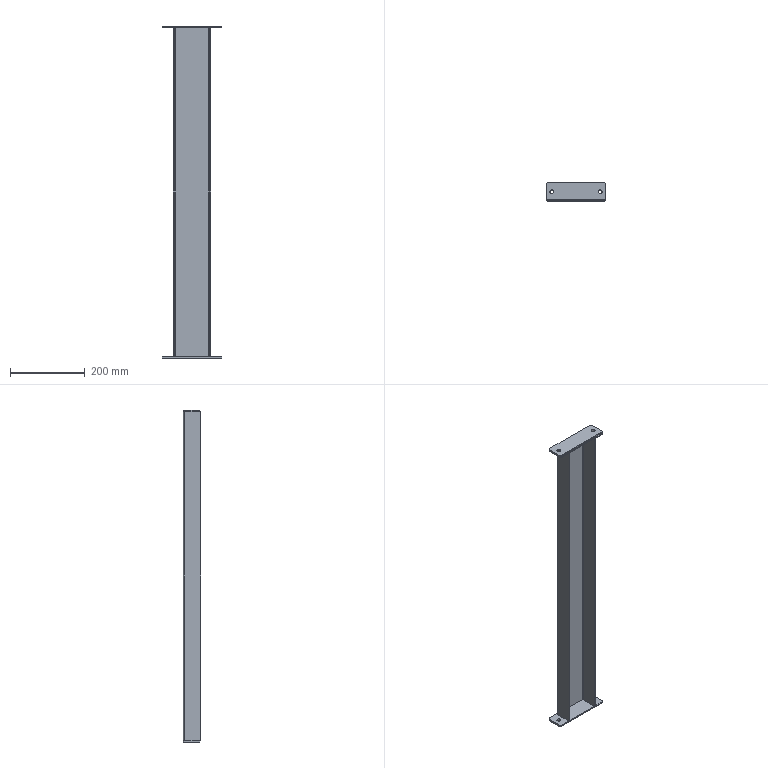Component | NX | TOP_BEAM | 3 solids | 42 faces | volume 403045 mm3 | plane 26 | cylinder 16 | commonest cylinder face diameters 10 x14 6 x2